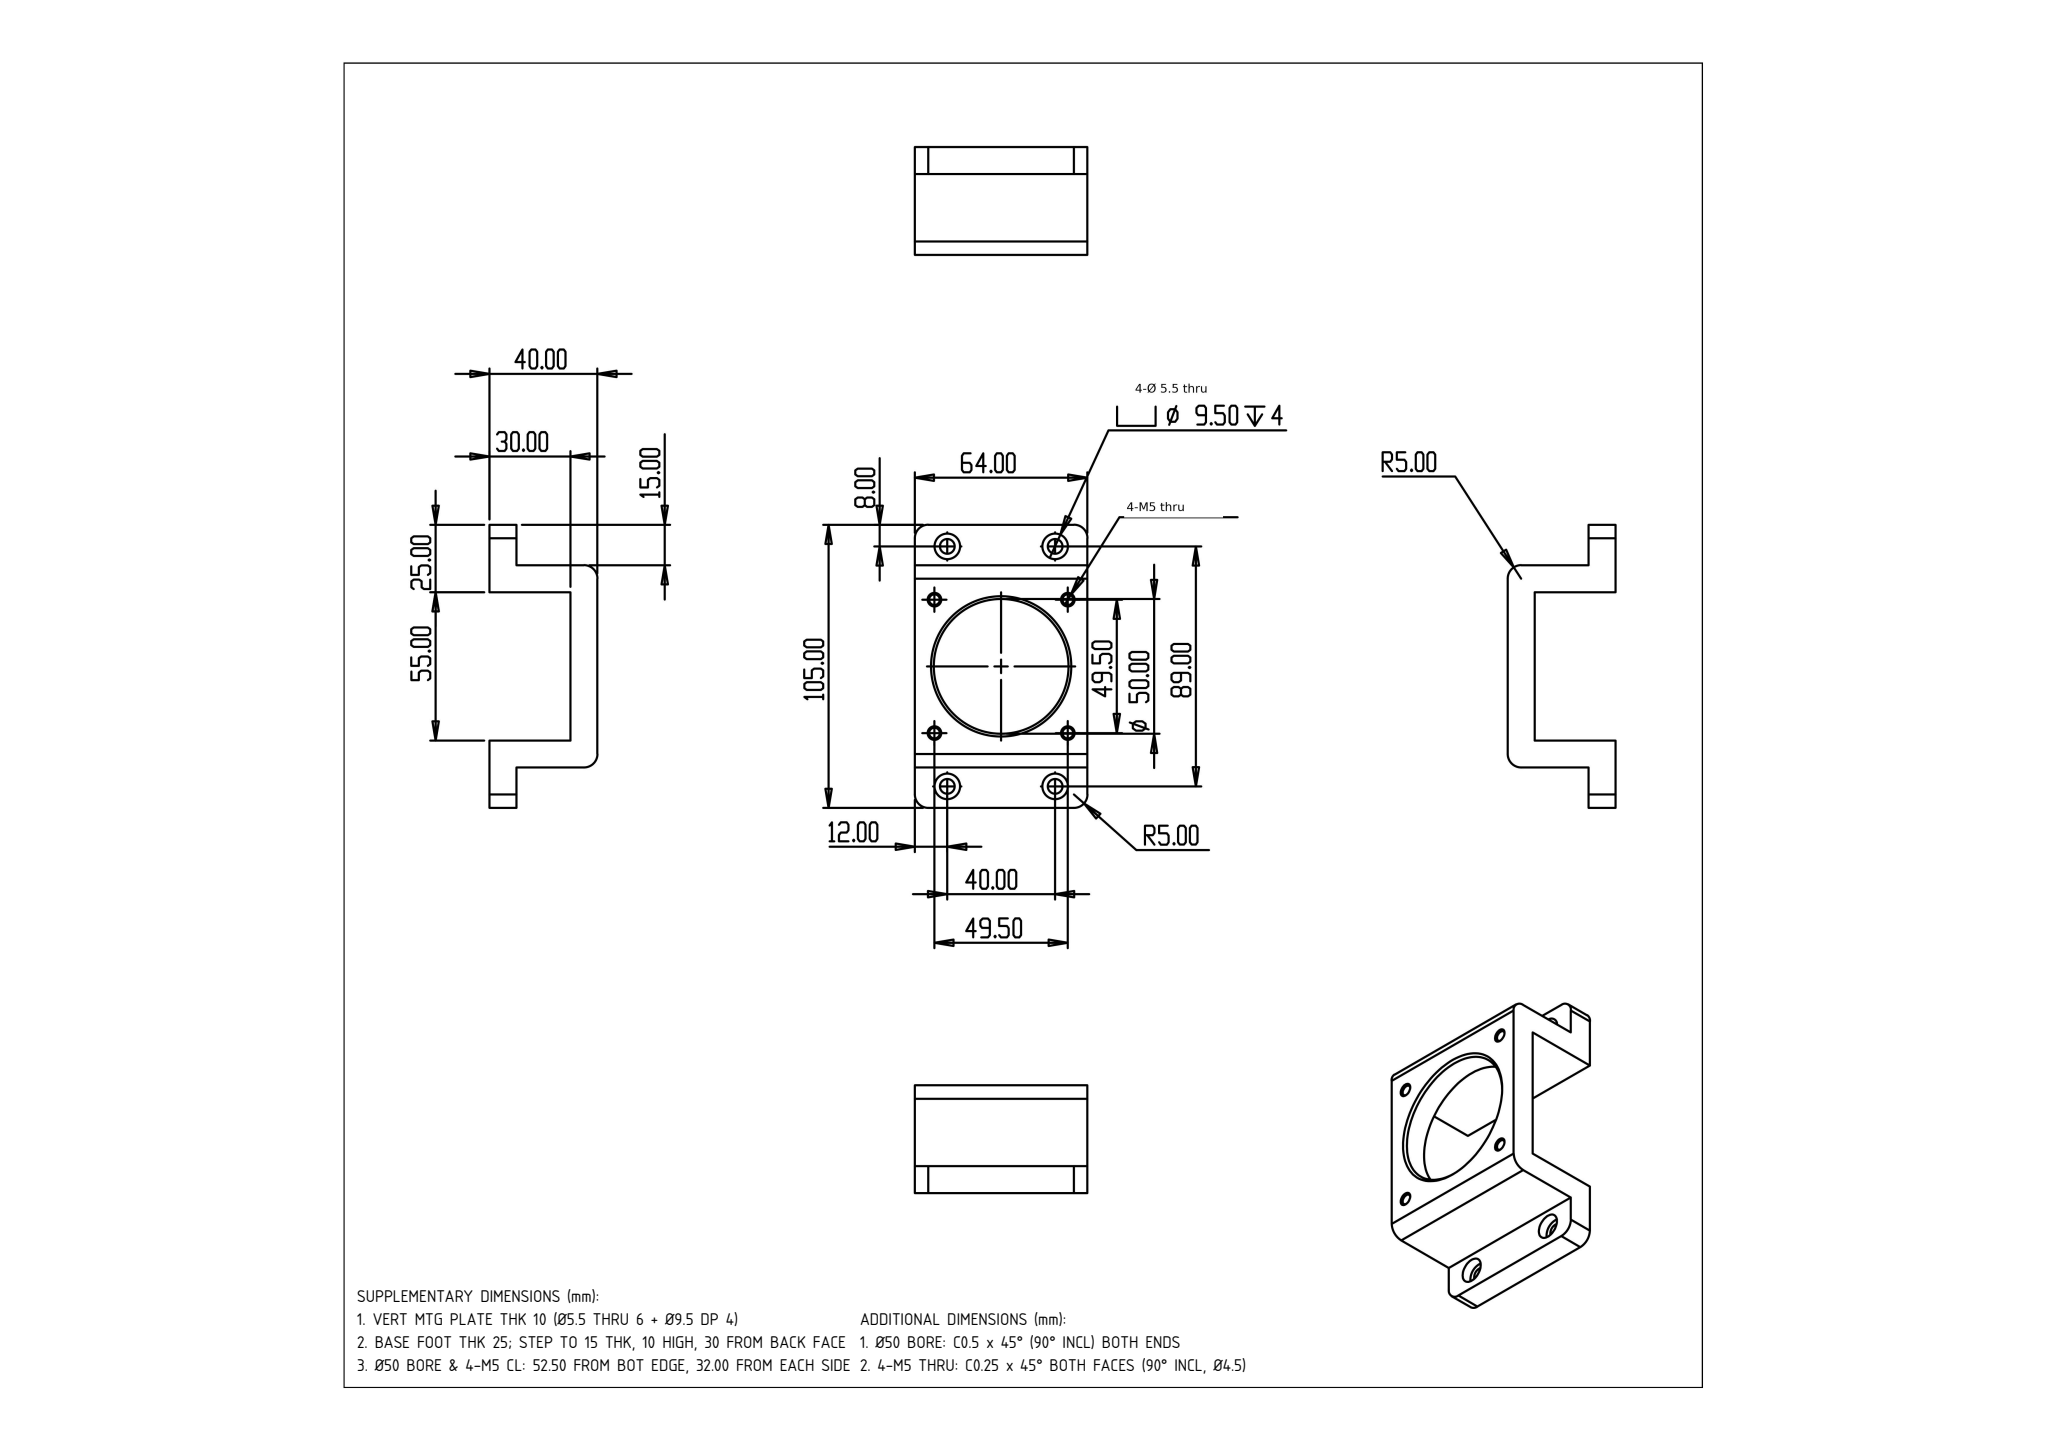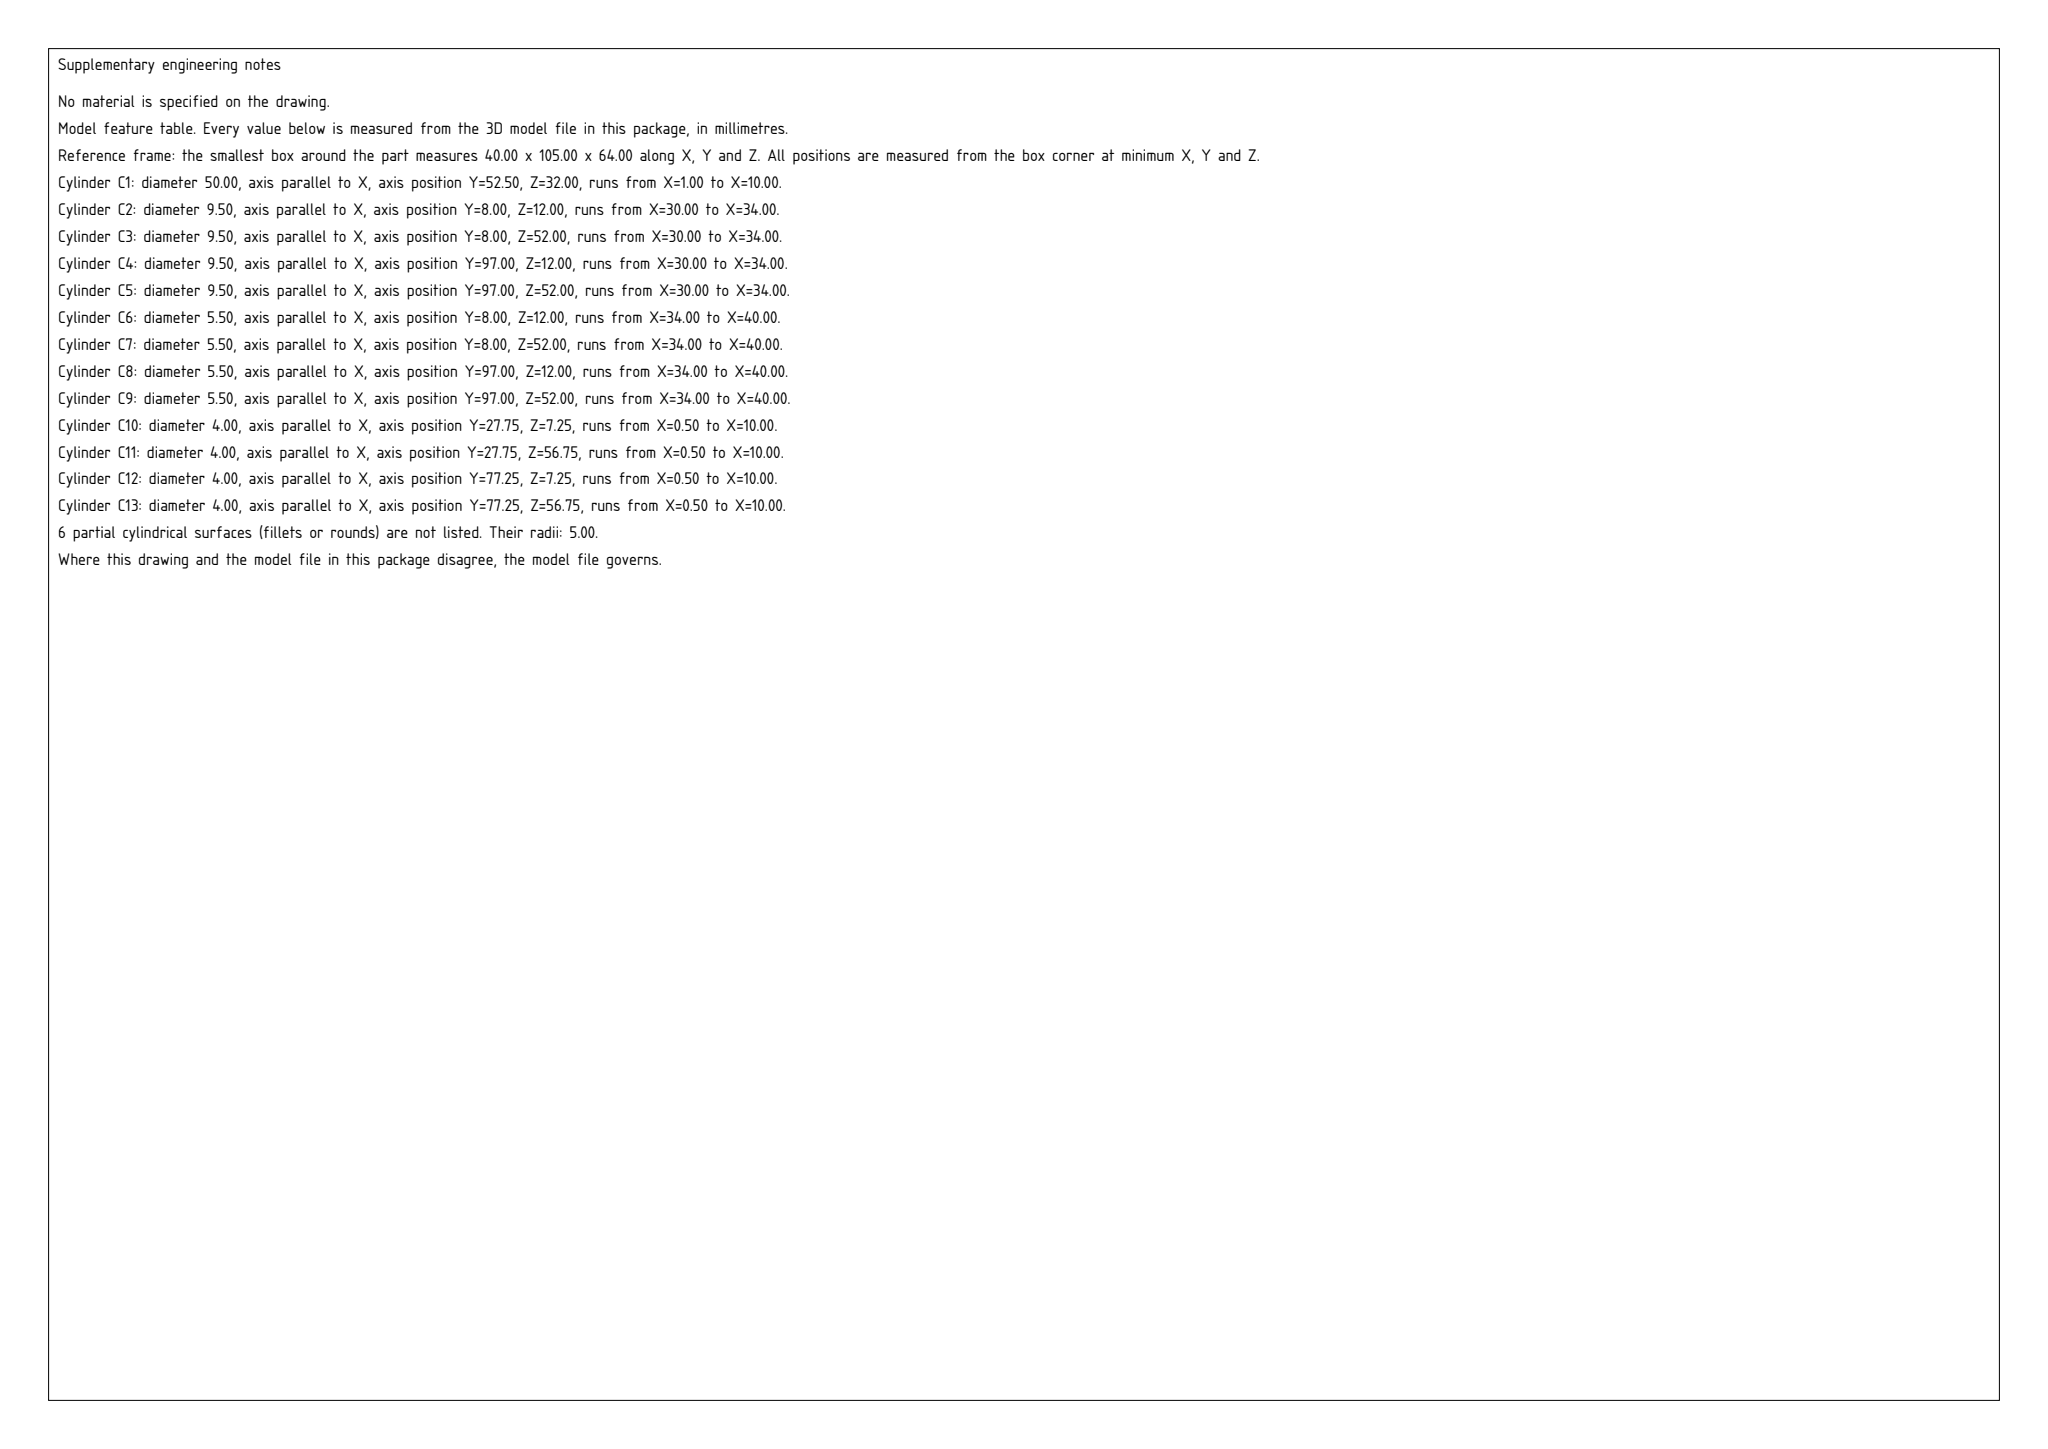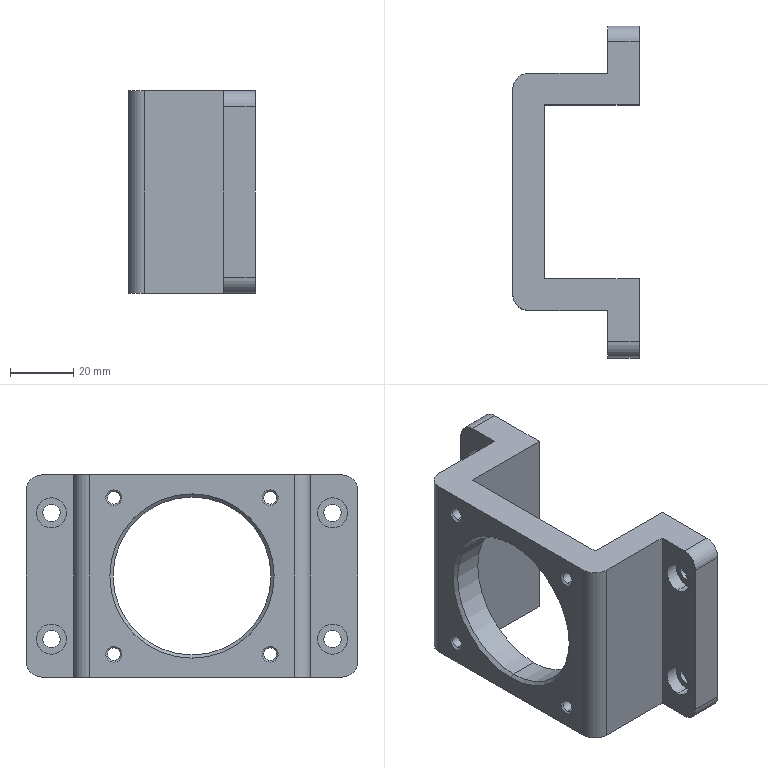Part | SolidWorks | mm | 1 solid | 60 faces | box 40 x 105 x 64 mm | volume 82770 mm3 | cylinder 32 | plane 18 | cone 10 | commonest cylinder face diameters 9.5 x8 4 x8 5.5 x8 10 x6 50 x2
build123d program:
from build123d import *

# Parameters (mm, degrees)
BOSS_EXTRUDE1_DEPTH = 64
FILLET1_R           = 5
CUT_EXTRUDE1_REACH  = 130.536
SKETCH2_R           = 2.75
SKETCH2_R_2         = 2
SKETCH2_R_3         = 25
SKETCH3_R           = 4.75
CUT_EXTRUDE2_DEPTH  = 4
CHAMFER1_SIZE       = 0.5
CHAMFER2_SIZE       = 1


with BuildPart() as part:
    # Sketch1 → Boss-Extrude1 (new body)
    with BuildSketch(Plane.XY):
        with BuildLine():
            Line((-30.45, 104.045), (-40.45, 104.045))
            Line((-40.45, 104.045), (-40.45, 99.045))
            Line((-40.45, 99.045), (-40.45, 89.045))
            Line((-40.45, 89.045), (-65.45, 89.045))
            ThreePointArc((-65.45, 89.045), (-68.986, 87.581), (-70.45, 84.045))
            Line((-70.45, 84.045), (-70.45, 19.045))
            ThreePointArc((-70.45, 19.045), (-68.986, 15.51), (-65.45, 14.045))
            Line((-65.45, 14.045), (-40.45, 14.045))
            Line((-40.45, 14.045), (-40.45, 4.045))
            Line((-40.45, 4.045), (-40.45, -0.9548))
            Line((-40.45, -0.9548), (-30.45, -0.9548))
            Line((-30.45, -0.9548), (-30.45, 4.045))
            Line((-30.45, 4.045), (-30.45, 24.045))
            Line((-30.45, 24.045), (-60.45, 24.045))
            Line((-60.45, 24.045), (-60.45, 79.045))
            Line((-60.45, 79.045), (-30.45, 79.045))
            Line((-30.45, 79.045), (-30.45, 99.045))
            Line((-30.45, 99.045), (-30.45, 104.045))
        make_face()
    extrude(amount=BOSS_EXTRUDE1_DEPTH)

    # Fillet1
    fillet1_edges = [part.edges().sort_by_distance(p)[0] for p in [
        (-35.45, -0.9548, 0),
        (-35.45, 104.045, 0),
        (-35.45, -0.9548, 64),
        (-35.45, 104.045, 64),
    ]]
    fillet(fillet1_edges, radius=FILLET1_R)

    # Sketch2 → Cut-Extrude1 (cut, up to next)
    with BuildSketch(Plane.ZY.offset(70.45), mode=Mode.PRIVATE) as cut_extrude1_sk1:
        with Locations(Location((52, 96.045, 0), (0, 0, 270))):
            Circle(SKETCH2_R)
    cut_extrude1_tool1 = extrude(cut_extrude1_sk1.sketch, amount=-CUT_EXTRUDE1_REACH, mode=Mode.PRIVATE) & part.part
    # Sketch2 → Cut-Extrude1 (cut, up to next)
    with BuildSketch(Plane.ZY.offset(70.45), mode=Mode.PRIVATE) as cut_extrude1_sk2:
        with Locations(Location((12, 96.045, 0), (0, 0, 270))):
            Circle(SKETCH2_R)
    cut_extrude1_tool2 = extrude(cut_extrude1_sk2.sketch, amount=-CUT_EXTRUDE1_REACH, mode=Mode.PRIVATE) & part.part
    # Sketch2 → Cut-Extrude1 (cut, up to next)
    with BuildSketch(Plane.ZY.offset(70.45), mode=Mode.PRIVATE) as cut_extrude1_sk3:
        with Locations((7.25, 76.295)):
            Circle(SKETCH2_R_2)
    cut_extrude1_tool3 = extrude(cut_extrude1_sk3.sketch, amount=-CUT_EXTRUDE1_REACH, mode=Mode.PRIVATE) & part.part
    # Sketch2 → Cut-Extrude1 (cut, up to next)
    with BuildSketch(Plane.ZY.offset(70.45), mode=Mode.PRIVATE) as cut_extrude1_sk4:
        with Locations((7.25, 26.795)):
            Circle(SKETCH2_R_2)
    cut_extrude1_tool4 = extrude(cut_extrude1_sk4.sketch, amount=-CUT_EXTRUDE1_REACH, mode=Mode.PRIVATE) & part.part
    # Sketch2 → Cut-Extrude1 (cut, up to next)
    with BuildSketch(Plane.ZY.offset(70.45), mode=Mode.PRIVATE) as cut_extrude1_sk5:
        with Locations(Location((12, 7.045, 0), (0, 0, 270))):
            Circle(SKETCH2_R)
    cut_extrude1_tool5 = extrude(cut_extrude1_sk5.sketch, amount=-CUT_EXTRUDE1_REACH, mode=Mode.PRIVATE) & part.part
    # Sketch2 → Cut-Extrude1 (cut, up to next)
    with BuildSketch(Plane.ZY.offset(70.45), mode=Mode.PRIVATE) as cut_extrude1_sk6:
        with Locations(Location((52, 7.045, 0), (0, 0, 270))):
            Circle(SKETCH2_R)
    cut_extrude1_tool6 = extrude(cut_extrude1_sk6.sketch, amount=-CUT_EXTRUDE1_REACH, mode=Mode.PRIVATE) & part.part
    # Sketch2 → Cut-Extrude1 (cut, up to next)
    with BuildSketch(Plane.ZY.offset(70.45), mode=Mode.PRIVATE) as cut_extrude1_sk7:
        with Locations((56.75, 26.795)):
            Circle(SKETCH2_R_2)
    cut_extrude1_tool7 = extrude(cut_extrude1_sk7.sketch, amount=-CUT_EXTRUDE1_REACH, mode=Mode.PRIVATE) & part.part
    # Sketch2 → Cut-Extrude1 (cut, up to next)
    with BuildSketch(Plane.ZY.offset(70.45), mode=Mode.PRIVATE) as cut_extrude1_sk8:
        with Locations((56.75, 76.295)):
            Circle(SKETCH2_R_2)
    cut_extrude1_tool8 = extrude(cut_extrude1_sk8.sketch, amount=-CUT_EXTRUDE1_REACH, mode=Mode.PRIVATE) & part.part
    # Sketch2 → Cut-Extrude1 (cut, up to next)
    with BuildSketch(Plane.ZY.offset(70.45), mode=Mode.PRIVATE) as cut_extrude1_sk9:
        with Locations((32, 51.545)):
            Circle(SKETCH2_R_3)
    cut_extrude1_tool9 = extrude(cut_extrude1_sk9.sketch, amount=-CUT_EXTRUDE1_REACH, mode=Mode.PRIVATE) & part.part
    add(cut_extrude1_tool1.solids().sort_by_distance((-70.45, 96.045, 52))[0], mode=Mode.SUBTRACT)
    add(cut_extrude1_tool2.solids().sort_by_distance((-70.45, 96.045, 12))[0], mode=Mode.SUBTRACT)
    add(cut_extrude1_tool3.solids().sort_by_distance((-70.45, 76.295, 7.25))[0], mode=Mode.SUBTRACT)
    add(cut_extrude1_tool4.solids().sort_by_distance((-70.45, 26.795, 7.25))[0], mode=Mode.SUBTRACT)
    add(cut_extrude1_tool5.solids().sort_by_distance((-70.45, 7.045, 12))[0], mode=Mode.SUBTRACT)
    add(cut_extrude1_tool6.solids().sort_by_distance((-70.45, 7.045, 52))[0], mode=Mode.SUBTRACT)
    add(cut_extrude1_tool7.solids().sort_by_distance((-70.45, 26.795, 56.75))[0], mode=Mode.SUBTRACT)
    add(cut_extrude1_tool8.solids().sort_by_distance((-70.45, 76.295, 56.75))[0], mode=Mode.SUBTRACT)
    add(cut_extrude1_tool9.solids().sort_by_distance((-70.45, 51.545, 32))[0], mode=Mode.SUBTRACT)

    # Sketch3 → Cut-Extrude2 (cut)
    with BuildSketch(Plane.ZY.offset(40.45)):
        with Locations((52, 96.045)):
            Circle(SKETCH3_R)
        with Locations((52, 7.045)):
            Circle(SKETCH3_R)
        with Locations((12, 7.045)):
            Circle(SKETCH3_R)
        with Locations((12, 96.045)):
            Circle(SKETCH3_R)
    extrude(amount=-CUT_EXTRUDE2_DEPTH, mode=Mode.SUBTRACT)

    # Chamfer1
    chamfer1_edges = [part.edges().sort_by_distance(p)[0] for p in [
        (-70.45, 76.295, 54.75),
        (-70.45, 26.795, 54.75),
        (-70.45, 76.295, 5.25),
        (-70.45, 26.795, 5.25),
    ]]
    chamfer(chamfer1_edges, length=CHAMFER1_SIZE)

    # Chamfer2
    chamfer2_edges = [part.edges().sort_by_distance(p)[0] for p in [
        (-70.45, 51.545, 7),
    ]]
    chamfer(chamfer2_edges, length=CHAMFER2_SIZE)


solid = part.part